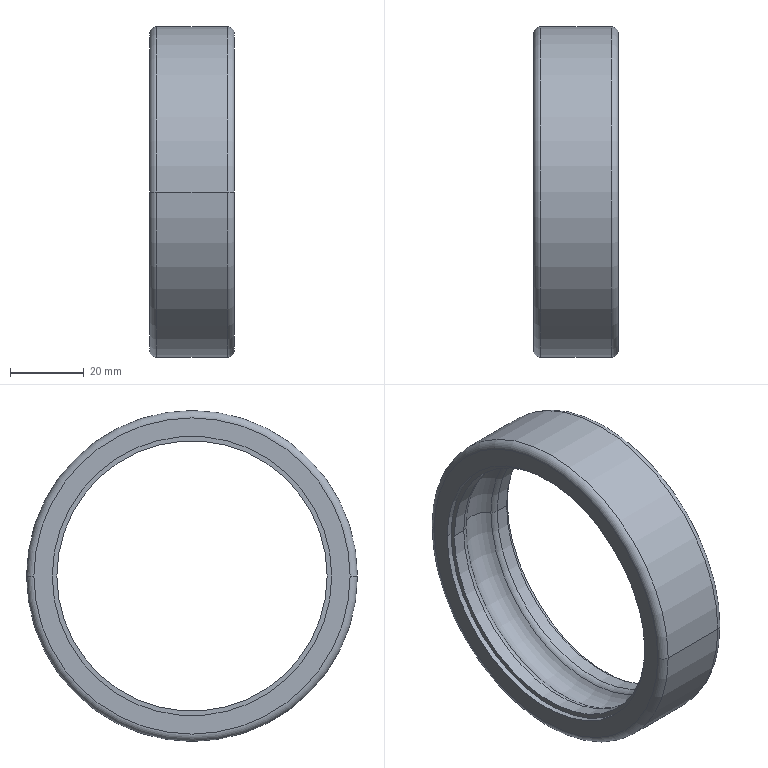Component | SolidWorks | 6308-OuterRing-1 | 1 solid | 24 faces | box 23.1 x 90 x 90 mm | volume 41581 mm3 | torus 10 | cylinder 10 | plane 4 | commonest cylinder face diameters 76 x4 73.5 x4 90 x2 | material AISI 304
build123d program:
from build123d import *

# Parameters (mm, degrees)
SKETCH1_R           = 45
SKETCH1_R_2         = 36.75
BOSS_EXTRUDE1_DEPTH = 11.55
FILLET1_R           = 2
SKETCH2_R           = 38
CUT_EXTRUDE1_DEPTH  = 1.5
SKETCH3_R           = 6
FILLET2_R           = 2


with BuildPart() as part:
    # Sketch1 → Boss-Extrude1 (new, symmetric)
    with BuildSketch(Plane.XY):
        Circle(SKETCH1_R)
        Circle(SKETCH1_R_2, mode=Mode.SUBTRACT)
    extrude(amount=BOSS_EXTRUDE1_DEPTH, both=True)

    # Fillet1
    fillet1_edges = [part.edges().sort_by_distance(p)[0] for p in [
        (-45, 0, -11.55),
        (-45, 0, 11.55),
    ]]
    fillet(fillet1_edges, radius=FILLET1_R)

    # Sketch2 → Cut-Extrude1 (cut)
    with BuildSketch(Plane.XY.offset(11.55)):
        Circle(SKETCH2_R)
    cut_extrude1 = extrude(amount=-CUT_EXTRUDE1_DEPTH, mode=Mode.SUBTRACT)

    # Mirror1: Cut-Extrude1 across plane
    add(cut_extrude1.mirror(Plane.XY), mode=Mode.SUBTRACT)

    # Sketch3 → Cut-Revolve1 (revolve, cut)
    with BuildSketch(Plane(origin=(0, 0, 0), x_dir=(0, 0, -1), z_dir=(1, 0, 0)), mode=Mode.PRIVATE) as cut_revolve1_sk:
        with Locations((0, 34)):
            Circle(SKETCH3_R)
    revolve(cut_revolve1_sk.sketch.rotate(Axis((0, 0, -32.915), (0, 0, 1)), 90), axis=Axis((0, 0, -32.915), (0, 0, 1)), mode=Mode.SUBTRACT)

    # Fillet2
    fillet2_edges = [part.edges().sort_by_distance(p)[0] for p in [
        (0, 36.75, 5.333),
        (0, -36.75, -5.333),
    ]]
    fillet(fillet2_edges, radius=FILLET2_R)


solid = part.part

# Placed as in the assembly
solid = solid.moved(Location((0, 136.117, 0), (0, 90, 0)))
STEP:
#1=COLOUR_RGB('',0.7922,0.8196,0.9333);
#2=FILL_AREA_STYLE_COLOUR('',#1);
#3=FILL_AREA_STYLE('',(#2));
#4=SURFACE_STYLE_FILL_AREA(#3);
#5=SURFACE_SIDE_STYLE('',(#4));
#6=SURFACE_STYLE_USAGE(.BOTH.,#5);
#7=PRESENTATION_STYLE_ASSIGNMENT((#6));
#8=CARTESIAN_POINT('',(0.1901,3.88,-0.));
#9=VERTEX_POINT('',#8);
#10=CARTESIAN_POINT('',(0.1901,6.838,-0.));
#11=VERTEX_POINT('',#10);
#12=CARTESIAN_POINT('',(0.1901,5.359,-0.));
#13=DIRECTION('',(1.,0.,0.));
#14=DIRECTION('',(-0.,1.,0.));
#15=AXIS2_PLACEMENT_3D('',#12,#13,#14);
#16=CIRCLE('',#15,1.479);
#17=EDGE_CURVE('',#9,#11,#16,.T.);
#18=ORIENTED_EDGE('',*,*,#17,.F.);
#19=CARTESIAN_POINT('',(0.2534,3.912,-0.));
#20=VERTEX_POINT('',#19);
#21=CARTESIAN_POINT('',(0.2534,3.833,-0.));
#22=DIRECTION('',(-0.,0.,-1.));
#23=DIRECTION('',(0.,1.,0.));
#24=AXIS2_PLACEMENT_3D('',#21,#22,#23);
#25=CIRCLE('',#24,0.07874);
#26=EDGE_CURVE('',#9,#20,#25,.T.);
#27=ORIENTED_EDGE('',*,*,#26,.T.);
#28=CARTESIAN_POINT('',(0.2534,6.806,-0.));
#29=VERTEX_POINT('',#28);
#30=CARTESIAN_POINT('',(0.2534,5.359,-0.));
#31=DIRECTION('',(-1.,-0.,-0.));
#32=DIRECTION('',(-0.,1.,0.));
#33=AXIS2_PLACEMENT_3D('',#30,#31,#32);
#34=CIRCLE('',#33,1.447);
#35=EDGE_CURVE('',#29,#20,#34,.T.);
#36=ORIENTED_EDGE('',*,*,#35,.F.);
#37=CARTESIAN_POINT('',(0.2534,6.885,-0.));
#38=DIRECTION('',(0.,-0.,1.));
#39=DIRECTION('',(0.,-1.,-0.));
#40=AXIS2_PLACEMENT_3D('',#37,#38,#39);
#41=CIRCLE('',#40,0.07874);
#42=EDGE_CURVE('',#11,#29,#41,.T.);
#43=ORIENTED_EDGE('',*,*,#42,.F.);
#44=EDGE_LOOP('',(#18,#27,#36,#43));
#45=FACE_OUTER_BOUND('',#44,.T.);
#46=CARTESIAN_POINT('',(0.2534,5.359,-0.));
#47=DIRECTION('',(-1.,-0.,-0.));
#48=DIRECTION('',(-0.,1.,0.));
#49=AXIS2_PLACEMENT_3D('',#46,#47,#48);
#50=TOROIDAL_SURFACE('',#49,1.526,0.07874);
#51=ADVANCED_FACE('',(#45),#50,.T.);
#52=CARTESIAN_POINT('',(-0.1901,6.838,-0.));
#53=VERTEX_POINT('',#52);
#54=CARTESIAN_POINT('',(-0.1901,3.88,-0.));
#55=VERTEX_POINT('',#54);
#56=CARTESIAN_POINT('',(-0.1901,5.359,-0.));
#57=DIRECTION('',(-1.,-0.,-0.));
#58=DIRECTION('',(0.,-1.,-0.));
#59=AXIS2_PLACEMENT_3D('',#56,#57,#58);
#60=CIRCLE('',#59,1.479);
#61=EDGE_CURVE('',#53,#55,#60,.T.);
#62=ORIENTED_EDGE('',*,*,#61,.F.);
#63=CARTESIAN_POINT('',(-0.2534,6.806,-0.));
#64=VERTEX_POINT('',#63);
#65=CARTESIAN_POINT('',(-0.2534,6.885,-0.));
#66=DIRECTION('',(0.,-0.,-1.));
#67=DIRECTION('',(0.,1.,-0.));
#68=AXIS2_PLACEMENT_3D('',#65,#66,#67);
#69=CIRCLE('',#68,0.07874);
#70=EDGE_CURVE('',#53,#64,#69,.T.);
#71=ORIENTED_EDGE('',*,*,#70,.T.);
#72=CARTESIAN_POINT('',(-0.2534,3.912,-0.));
#73=VERTEX_POINT('',#72);
#74=CARTESIAN_POINT('',(-0.2534,5.359,-0.));
#75=DIRECTION('',(1.,0.,0.));
#76=DIRECTION('',(0.,-1.,-0.));
#77=AXIS2_PLACEMENT_3D('',#74,#75,#76);
#78=CIRCLE('',#77,1.447);
#79=EDGE_CURVE('',#73,#64,#78,.T.);
#80=ORIENTED_EDGE('',*,*,#79,.F.);
#81=CARTESIAN_POINT('',(-0.2534,3.833,-0.));
#82=DIRECTION('',(0.,-0.,1.));
#83=DIRECTION('',(0.,-1.,-0.));
#84=AXIS2_PLACEMENT_3D('',#81,#82,#83);
#85=CIRCLE('',#84,0.07874);
#86=EDGE_CURVE('',#55,#73,#85,.T.);
#87=ORIENTED_EDGE('',*,*,#86,.F.);
#88=EDGE_LOOP('',(#62,#71,#80,#87));
#89=FACE_OUTER_BOUND('',#88,.T.);
#90=CARTESIAN_POINT('',(-0.2534,5.359,-0.));
#91=DIRECTION('',(1.,0.,0.));
#92=DIRECTION('',(0.,-1.,-0.));
#93=AXIS2_PLACEMENT_3D('',#90,#91,#92);
#94=TOROIDAL_SURFACE('',#93,1.526,0.07874);
#95=ADVANCED_FACE('',(#89),#94,.T.);
#96=CARTESIAN_POINT('',(0.1901,5.359,-0.));
#97=DIRECTION('',(1.,0.,0.));
#98=DIRECTION('',(-0.,1.,0.));
#99=AXIS2_PLACEMENT_3D('',#96,#97,#98);
#100=CIRCLE('',#99,1.479);
#101=EDGE_CURVE('',#11,#9,#100,.T.);
#102=ORIENTED_EDGE('',*,*,#101,.T.);
#103=CARTESIAN_POINT('',(-0.,4.02,-0.));
#104=DIRECTION('',(-0.,0.,-1.));
#105=DIRECTION('',(0.,1.,0.));
#106=AXIS2_PLACEMENT_3D('',#103,#104,#105);
#107=CIRCLE('',#106,0.2362);
#108=EDGE_CURVE('',#9,#55,#107,.T.);
#109=ORIENTED_EDGE('',*,*,#108,.T.);
#110=CARTESIAN_POINT('',(-0.1901,5.359,-0.));
#111=DIRECTION('',(-1.,-0.,-0.));
#112=DIRECTION('',(0.,-1.,-0.));
#113=AXIS2_PLACEMENT_3D('',#110,#111,#112);
#114=CIRCLE('',#113,1.479);
#115=EDGE_CURVE('',#55,#53,#114,.T.);
#116=ORIENTED_EDGE('',*,*,#115,.T.);
#117=CARTESIAN_POINT('',(-0.,6.698,-0.));
#118=DIRECTION('',(0.,-0.,1.));
#119=DIRECTION('',(0.,-1.,-0.));
#120=AXIS2_PLACEMENT_3D('',#117,#118,#119);
#121=CIRCLE('',#120,0.2362);
#122=EDGE_CURVE('',#11,#53,#121,.T.);
#123=ORIENTED_EDGE('',*,*,#122,.F.);
#124=EDGE_LOOP('',(#102,#109,#116,#123));
#125=FACE_OUTER_BOUND('',#124,.T.);
#126=CARTESIAN_POINT('',(-0.,5.359,-0.));
#127=DIRECTION('',(-1.,-0.,-0.));
#128=DIRECTION('',(-0.,1.,0.));
#129=AXIS2_PLACEMENT_3D('',#126,#127,#128);
#130=TOROIDAL_SURFACE('',#129,1.339,0.2362);
#131=ADVANCED_FACE('',(#125),#130,.F.);
#132=CARTESIAN_POINT('',(-0.3957,6.855,-0.));
#133=VERTEX_POINT('',#132);
#134=CARTESIAN_POINT('',(-0.3957,3.863,-0.));
#135=VERTEX_POINT('',#134);
#136=CARTESIAN_POINT('',(-0.3957,5.359,-0.));
#137=DIRECTION('',(1.,0.,0.));
#138=DIRECTION('',(0.,-1.,-0.));
#139=AXIS2_PLACEMENT_3D('',#136,#137,#138);
#140=CIRCLE('',#139,1.496);
#141=EDGE_CURVE('',#133,#135,#140,.T.);
#142=ORIENTED_EDGE('',*,*,#141,.T.);
#143=CARTESIAN_POINT('',(-0.4547,3.863,-0.));
#144=VERTEX_POINT('',#143);
#145=CARTESIAN_POINT('',(-0.3957,3.863,-0.));
#146=DIRECTION('',(-1.,-0.,-0.));
#147=VECTOR('',#146,39.37);
#148=LINE('',#145,#147);
#149=EDGE_CURVE('',#135,#144,#148,.T.);
#150=ORIENTED_EDGE('',*,*,#149,.T.);
#151=CARTESIAN_POINT('',(-0.4547,6.855,-0.));
#152=VERTEX_POINT('',#151);
#153=CARTESIAN_POINT('',(-0.4547,5.359,-0.));
#154=DIRECTION('',(1.,0.,0.));
#155=DIRECTION('',(0.,-1.,-0.));
#156=AXIS2_PLACEMENT_3D('',#153,#154,#155);
#157=CIRCLE('',#156,1.496);
#158=EDGE_CURVE('',#152,#144,#157,.T.);
#159=ORIENTED_EDGE('',*,*,#158,.F.);
#160=CARTESIAN_POINT('',(-0.3957,6.855,-0.));
#161=DIRECTION('',(-1.,-0.,-0.));
#162=VECTOR('',#161,39.37);
#163=LINE('',#160,#162);
#164=EDGE_CURVE('',#133,#152,#163,.T.);
#165=ORIENTED_EDGE('',*,*,#164,.F.);
#166=EDGE_LOOP('',(#142,#150,#159,#165));
#167=FACE_OUTER_BOUND('',#166,.T.);
#168=CARTESIAN_POINT('',(-0.3957,5.359,-0.));
#169=DIRECTION('',(-1.,-0.,-0.));
#170=DIRECTION('',(-0.,1.,0.));
#171=AXIS2_PLACEMENT_3D('',#168,#169,#170);
#172=CYLINDRICAL_SURFACE('',#171,1.496);
#173=ADVANCED_FACE('',(#167),#172,.F.);
#174=CARTESIAN_POINT('',(0.3957,6.855,-0.));
#175=VERTEX_POINT('',#174);
#176=CARTESIAN_POINT('',(0.3957,3.863,-0.));
#177=VERTEX_POINT('',#176);
#178=CARTESIAN_POINT('',(0.3957,5.359,-0.));
#179=DIRECTION('',(1.,0.,0.));
#180=DIRECTION('',(0.,-1.,-0.));
#181=AXIS2_PLACEMENT_3D('',#178,#179,#180);
#182=CIRCLE('',#181,1.496);
#183=EDGE_CURVE('',#175,#177,#182,.T.);
#184=ORIENTED_EDGE('',*,*,#183,.F.);
#185=CARTESIAN_POINT('',(0.4547,6.855,-0.));
#186=VERTEX_POINT('',#185);
#187=CARTESIAN_POINT('',(0.3957,6.855,-0.));
#188=DIRECTION('',(1.,0.,0.));
#189=VECTOR('',#188,39.37);
#190=LINE('',#187,#189);
#191=EDGE_CURVE('',#175,#186,#190,.T.);
#192=ORIENTED_EDGE('',*,*,#191,.T.);
#193=CARTESIAN_POINT('',(0.4547,3.863,-0.));
#194=VERTEX_POINT('',#193);
#195=CARTESIAN_POINT('',(0.4547,5.359,-0.));
#196=DIRECTION('',(1.,0.,0.));
#197=DIRECTION('',(0.,-1.,-0.));
#198=AXIS2_PLACEMENT_3D('',#195,#196,#197);
#199=CIRCLE('',#198,1.496);
#200=EDGE_CURVE('',#186,#194,#199,.T.);
#201=ORIENTED_EDGE('',*,*,#200,.T.);
#202=CARTESIAN_POINT('',(0.3957,3.863,-0.));
#203=DIRECTION('',(1.,0.,0.));
#204=VECTOR('',#203,39.37);
#205=LINE('',#202,#204);
#206=EDGE_CURVE('',#177,#194,#205,.T.);
#207=ORIENTED_EDGE('',*,*,#206,.F.);
#208=EDGE_LOOP('',(#184,#192,#201,#207));
#209=FACE_OUTER_BOUND('',#208,.T.);
#210=CARTESIAN_POINT('',(0.3957,5.359,-0.));
#211=DIRECTION('',(1.,0.,0.));
#212=DIRECTION('',(0.,-1.,-0.));
#213=AXIS2_PLACEMENT_3D('',#210,#211,#212);
#214=CYLINDRICAL_SURFACE('',#213,1.496);
#215=ADVANCED_FACE('',(#209),#214,.F.);
#216=CARTESIAN_POINT('',(0.376,7.131,-0.));
#217=VERTEX_POINT('',#216);
#218=CARTESIAN_POINT('',(0.376,3.587,-0.));
#219=VERTEX_POINT('',#218);
#220=CARTESIAN_POINT('',(0.376,5.359,-0.));
#221=DIRECTION('',(-1.,-0.,-0.));
#222=DIRECTION('',(0.,-1.,-0.));
#223=AXIS2_PLACEMENT_3D('',#220,#221,#222);
#224=CIRCLE('',#223,1.772);
#225=EDGE_CURVE('',#217,#219,#224,.T.);
#226=ORIENTED_EDGE('',*,*,#225,.F.);
#227=CARTESIAN_POINT('',(0.4547,7.052,-0.));
#228=VERTEX_POINT('',#227);
#229=CARTESIAN_POINT('',(0.376,7.052,-0.));
#230=DIRECTION('',(0.,-0.,-1.));
#231=DIRECTION('',(0.,1.,-0.));
#232=AXIS2_PLACEMENT_3D('',#229,#230,#231);
#233=CIRCLE('',#232,0.07874);
#234=EDGE_CURVE('',#217,#228,#233,.T.);
#235=ORIENTED_EDGE('',*,*,#234,.T.);
#236=CARTESIAN_POINT('',(0.4547,3.666,-0.));
#237=VERTEX_POINT('',#236);
#238=CARTESIAN_POINT('',(0.4547,5.359,-0.));
#239=DIRECTION('',(1.,0.,0.));
#240=DIRECTION('',(0.,-1.,-0.));
#241=AXIS2_PLACEMENT_3D('',#238,#239,#240);
#242=CIRCLE('',#241,1.693);
#243=EDGE_CURVE('',#237,#228,#242,.T.);
#244=ORIENTED_EDGE('',*,*,#243,.F.);
#245=CARTESIAN_POINT('',(0.376,3.666,-0.));
#246=DIRECTION('',(0.,-0.,1.));
#247=DIRECTION('',(0.,-1.,-0.));
#248=AXIS2_PLACEMENT_3D('',#245,#246,#247);
#249=CIRCLE('',#248,0.07874);
#250=EDGE_CURVE('',#219,#237,#249,.T.);
#251=ORIENTED_EDGE('',*,*,#250,.F.);
#252=EDGE_LOOP('',(#226,#235,#244,#251));
#253=FACE_OUTER_BOUND('',#252,.T.);
#254=CARTESIAN_POINT('',(0.376,5.359,-0.));
#255=DIRECTION('',(1.,0.,0.));
#256=DIRECTION('',(0.,-1.,-0.));
#257=AXIS2_PLACEMENT_3D('',#254,#255,#256);
#258=TOROIDAL_SURFACE('',#257,1.693,0.07874);
#259=ADVANCED_FACE('',(#253),#258,.T.);
#260=CARTESIAN_POINT('',(-0.4547,7.052,-0.));
#261=VERTEX_POINT('',#260);
#262=CARTESIAN_POINT('',(-0.4547,3.666,-0.));
#263=VERTEX_POINT('',#262);
#264=CARTESIAN_POINT('',(-0.4547,5.359,-0.));
#265=DIRECTION('',(-1.,-0.,-0.));
#266=DIRECTION('',(0.,-1.,-0.));
#267=AXIS2_PLACEMENT_3D('',#264,#265,#266);
#268=CIRCLE('',#267,1.693);
#269=EDGE_CURVE('',#261,#263,#268,.T.);
#270=ORIENTED_EDGE('',*,*,#269,.F.);
#271=CARTESIAN_POINT('',(-0.376,7.131,-0.));
#272=VERTEX_POINT('',#271);
#273=CARTESIAN_POINT('',(-0.376,7.052,-0.));
#274=DIRECTION('',(0.,-0.,-1.));
#275=DIRECTION('',(0.,1.,-0.));
#276=AXIS2_PLACEMENT_3D('',#273,#274,#275);
#277=CIRCLE('',#276,0.07874);
#278=EDGE_CURVE('',#261,#272,#277,.T.);
#279=ORIENTED_EDGE('',*,*,#278,.T.);
#280=CARTESIAN_POINT('',(-0.376,3.587,-0.));
#281=VERTEX_POINT('',#280);
#282=CARTESIAN_POINT('',(-0.376,5.359,-0.));
#283=DIRECTION('',(1.,0.,0.));
#284=DIRECTION('',(0.,-1.,-0.));
#285=AXIS2_PLACEMENT_3D('',#282,#283,#284);
#286=CIRCLE('',#285,1.772);
#287=EDGE_CURVE('',#281,#272,#286,.T.);
#288=ORIENTED_EDGE('',*,*,#287,.F.);
#289=CARTESIAN_POINT('',(-0.376,3.666,-0.));
#290=DIRECTION('',(0.,-0.,1.));
#291=DIRECTION('',(0.,-1.,-0.));
#292=AXIS2_PLACEMENT_3D('',#289,#290,#291);
#293=CIRCLE('',#292,0.07874);
#294=EDGE_CURVE('',#263,#281,#293,.T.);
#295=ORIENTED_EDGE('',*,*,#294,.F.);
#296=EDGE_LOOP('',(#270,#279,#288,#295));
#297=FACE_OUTER_BOUND('',#296,.T.);
#298=CARTESIAN_POINT('',(-0.376,5.359,-0.));
#299=DIRECTION('',(1.,0.,0.));
#300=DIRECTION('',(0.,-1.,-0.));
#301=AXIS2_PLACEMENT_3D('',#298,#299,#300);
#302=TOROIDAL_SURFACE('',#301,1.693,0.07874);
#303=ADVANCED_FACE('',(#297),#302,.T.);
#304=ORIENTED_EDGE('',*,*,#225,.T.);
#305=CARTESIAN_POINT('',(0.4547,3.587,-0.));
#306=DIRECTION('',(-1.,-0.,-0.));
#307=VECTOR('',#306,39.37);
#308=LINE('',#305,#307);
#309=EDGE_CURVE('',#219,#281,#308,.T.);
#310=ORIENTED_EDGE('',*,*,#309,.T.);
#311=ORIENTED_EDGE('',*,*,#287,.T.);
#312=CARTESIAN_POINT('',(0.4547,7.131,-0.));
#313=DIRECTION('',(-1.,-0.,-0.));
#314=VECTOR('',#313,39.37);
#315=LINE('',#312,#314);
#316=EDGE_CURVE('',#217,#272,#315,.T.);
#317=ORIENTED_EDGE('',*,*,#316,.F.);
#318=EDGE_LOOP('',(#304,#310,#311,#317));
#319=FACE_OUTER_BOUND('',#318,.T.);
#320=CARTESIAN_POINT('',(0.4547,5.359,-0.));
#321=DIRECTION('',(-1.,-0.,-0.));
#322=DIRECTION('',(-0.,1.,0.));
#323=AXIS2_PLACEMENT_3D('',#320,#321,#322);
#324=CYLINDRICAL_SURFACE('',#323,1.772);
#325=ADVANCED_FACE('',(#319),#324,.T.);
#326=CARTESIAN_POINT('',(0.3957,6.806,-0.));
#327=VERTEX_POINT('',#326);
#328=CARTESIAN_POINT('',(0.3957,3.912,-0.));
#329=VERTEX_POINT('',#328);
#330=CARTESIAN_POINT('',(0.3957,5.359,-0.));
#331=DIRECTION('',(1.,0.,0.));
#332=DIRECTION('',(0.,-1.,-0.));
#333=AXIS2_PLACEMENT_3D('',#330,#331,#332);
#334=CIRCLE('',#333,1.447);
#335=EDGE_CURVE('',#327,#329,#334,.T.);
#336=ORIENTED_EDGE('',*,*,#335,.T.);
#337=CARTESIAN_POINT('',(0.4547,3.912,-0.));
#338=DIRECTION('',(-1.,-0.,-0.));
#339=VECTOR('',#338,39.37);
#340=LINE('',#337,#339);
#341=EDGE_CURVE('',#329,#20,#340,.T.);
#342=ORIENTED_EDGE('',*,*,#341,.T.);
#343=CARTESIAN_POINT('',(0.2534,5.359,-0.));
#344=DIRECTION('',(-1.,-0.,-0.));
#345=DIRECTION('',(-0.,1.,0.));
#346=AXIS2_PLACEMENT_3D('',#343,#344,#345);
#347=CIRCLE('',#346,1.447);
#348=EDGE_CURVE('',#20,#29,#347,.T.);
#349=ORIENTED_EDGE('',*,*,#348,.T.);
#350=CARTESIAN_POINT('',(0.4547,6.806,-0.));
#351=DIRECTION('',(-1.,-0.,-0.));
#352=VECTOR('',#351,39.37);
#353=LINE('',#350,#352);
#354=EDGE_CURVE('',#327,#29,#353,.T.);
#355=ORIENTED_EDGE('',*,*,#354,.F.);
#356=EDGE_LOOP('',(#336,#342,#349,#355));
#357=FACE_OUTER_BOUND('',#356,.T.);
#358=CARTESIAN_POINT('',(0.4547,5.359,-0.));
#359=DIRECTION('',(-1.,-0.,-0.));
#360=DIRECTION('',(-0.,1.,0.));
#361=AXIS2_PLACEMENT_3D('',#358,#359,#360);
#362=CYLINDRICAL_SURFACE('',#361,1.447);
#363=ADVANCED_FACE('',(#357),#362,.F.);
#364=CARTESIAN_POINT('',(-0.2534,5.359,-0.));
#365=DIRECTION('',(1.,0.,0.));
#366=DIRECTION('',(0.,-1.,-0.));
#367=AXIS2_PLACEMENT_3D('',#364,#365,#366);
#368=CIRCLE('',#367,1.447);
#369=EDGE_CURVE('',#64,#73,#368,.T.);
#370=ORIENTED_EDGE('',*,*,#369,.T.);
#371=CARTESIAN_POINT('',(-0.3957,3.912,-0.));
#372=VERTEX_POINT('',#371);
#373=CARTESIAN_POINT('',(0.4547,3.912,-0.));
#374=DIRECTION('',(-1.,-0.,-0.));
#375=VECTOR('',#374,39.37);
#376=LINE('',#373,#375);
#377=EDGE_CURVE('',#73,#372,#376,.T.);
#378=ORIENTED_EDGE('',*,*,#377,.T.);
#379=CARTESIAN_POINT('',(-0.3957,6.806,-0.));
#380=VERTEX_POINT('',#379);
#381=CARTESIAN_POINT('',(-0.3957,5.359,-0.));
#382=DIRECTION('',(-1.,-0.,-0.));
#383=DIRECTION('',(-0.,1.,0.));
#384=AXIS2_PLACEMENT_3D('',#381,#382,#383);
#385=CIRCLE('',#384,1.447);
#386=EDGE_CURVE('',#372,#380,#385,.T.);
#387=ORIENTED_EDGE('',*,*,#386,.T.);
#388=CARTESIAN_POINT('',(0.4547,6.806,-0.));
#389=DIRECTION('',(-1.,-0.,-0.));
#390=VECTOR('',#389,39.37);
#391=LINE('',#388,#390);
#392=EDGE_CURVE('',#64,#380,#391,.T.);
#393=ORIENTED_EDGE('',*,*,#392,.F.);
#394=EDGE_LOOP('',(#370,#378,#387,#393));
#395=FACE_OUTER_BOUND('',#394,.T.);
#396=CARTESIAN_POINT('',(0.4547,5.359,-0.));
#397=DIRECTION('',(-1.,-0.,-0.));
#398=DIRECTION('',(-0.,1.,0.));
#399=AXIS2_PLACEMENT_3D('',#396,#397,#398);
#400=CYLINDRICAL_SURFACE('',#399,1.447);
#401=ADVANCED_FACE('',(#395),#400,.F.);
#402=ORIENTED_EDGE('',*,*,#377,.F.);
#403=ORIENTED_EDGE('',*,*,#79,.T.);
#404=ORIENTED_EDGE('',*,*,#392,.T.);
#405=CARTESIAN_POINT('',(-0.3957,5.359,-0.));
#406=DIRECTION('',(-1.,-0.,-0.));
#407=DIRECTION('',(-0.,1.,0.));
#408=AXIS2_PLACEMENT_3D('',#405,#406,#407);
#409=CIRCLE('',#408,1.447);
#410=EDGE_CURVE('',#380,#372,#409,.T.);
#411=ORIENTED_EDGE('',*,*,#410,.T.);
#412=EDGE_LOOP('',(#402,#403,#404,#411));
#413=FACE_OUTER_BOUND('',#412,.T.);
#414=CARTESIAN_POINT('',(0.4547,5.359,-0.));
#415=DIRECTION('',(-1.,-0.,-0.));
#416=DIRECTION('',(-0.,1.,0.));
#417=AXIS2_PLACEMENT_3D('',#414,#415,#416);
#418=CYLINDRICAL_SURFACE('',#417,1.447);
#419=ADVANCED_FACE('',(#413),#418,.F.);
#420=ORIENTED_EDGE('',*,*,#341,.F.);
#421=CARTESIAN_POINT('',(0.3957,5.359,-0.));
#422=DIRECTION('',(1.,0.,0.));
#423=DIRECTION('',(0.,-1.,-0.));
#424=AXIS2_PLACEMENT_3D('',#421,#422,#423);
#425=CIRCLE('',#424,1.447);
#426=EDGE_CURVE('',#329,#327,#425,.T.);
#427=ORIENTED_EDGE('',*,*,#426,.T.);
#428=ORIENTED_EDGE('',*,*,#354,.T.);
#429=ORIENTED_EDGE('',*,*,#35,.T.);
#430=EDGE_LOOP('',(#420,#427,#428,#429));
#431=FACE_OUTER_BOUND('',#430,.T.);
#432=CARTESIAN_POINT('',(0.4547,5.359,-0.));
#433=DIRECTION('',(-1.,-0.,-0.));
#434=DIRECTION('',(-0.,1.,0.));
#435=AXIS2_PLACEMENT_3D('',#432,#433,#434);
#436=CYLINDRICAL_SURFACE('',#435,1.447);
#437=ADVANCED_FACE('',(#431),#436,.F.);
#438=CARTESIAN_POINT('',(0.4547,5.359,-0.));
#439=DIRECTION('',(1.,0.,0.));
#440=DIRECTION('',(0.,-1.,-0.));
#441=AXIS2_PLACEMENT_3D('',#438,#439,#440);
#442=CIRCLE('',#441,1.496);
#443=EDGE_CURVE('',#194,#186,#442,.T.);
#444=ORIENTED_EDGE('',*,*,#443,.F.);
#445=ORIENTED_EDGE('',*,*,#200,.F.);
#446=EDGE_LOOP('',(#444,#445));
#447=FACE_BOUND('',#446,.T.);
#448=ORIENTED_EDGE('',*,*,#243,.T.);
#449=CARTESIAN_POINT('',(0.4547,5.359,-0.));
#450=DIRECTION('',(1.,0.,0.));
#451=DIRECTION('',(0.,-1.,-0.));
#452=AXIS2_PLACEMENT_3D('',#449,#450,#451);
#453=CIRCLE('',#452,1.693);
#454=EDGE_CURVE('',#228,#237,#453,.T.);
#455=ORIENTED_EDGE('',*,*,#454,.T.);
#456=EDGE_LOOP('',(#448,#455));
#457=FACE_OUTER_BOUND('',#456,.T.);
#458=CARTESIAN_POINT('',(0.4547,5.359,-0.));
#459=DIRECTION('',(1.,0.,0.));
#460=DIRECTION('',(0.,-1.,-0.));
#461=AXIS2_PLACEMENT_3D('',#458,#459,#460);
#462=PLANE('',#461);
#463=ADVANCED_FACE('',(#447,#457),#462,.T.);
#464=ORIENTED_EDGE('',*,*,#158,.T.);
#465=CARTESIAN_POINT('',(-0.4547,5.359,-0.));
#466=DIRECTION('',(1.,0.,0.));
#467=DIRECTION('',(0.,-1.,-0.));
#468=AXIS2_PLACEMENT_3D('',#465,#466,#467);
#469=CIRCLE('',#468,1.496);
#470=EDGE_CURVE('',#144,#152,#469,.T.);
#471=ORIENTED_EDGE('',*,*,#470,.T.);
#472=EDGE_LOOP('',(#464,#471));
#473=FACE_BOUND('',#472,.T.);
#474=CARTESIAN_POINT('',(-0.4547,5.359,-0.));
#475=DIRECTION('',(-1.,-0.,-0.));
#476=DIRECTION('',(0.,-1.,-0.));
#477=AXIS2_PLACEMENT_3D('',#474,#475,#476);
#478=CIRCLE('',#477,1.693);
#479=EDGE_CURVE('',#263,#261,#478,.T.);
#480=ORIENTED_EDGE('',*,*,#479,.T.);
#481=ORIENTED_EDGE('',*,*,#269,.T.);
#482=EDGE_LOOP('',(#480,#481));
#483=FACE_OUTER_BOUND('',#482,.T.);
#484=CARTESIAN_POINT('',(-0.4547,5.359,-0.));
#485=DIRECTION('',(1.,0.,0.));
#486=DIRECTION('',(0.,-1.,-0.));
#487=AXIS2_PLACEMENT_3D('',#484,#485,#486);
#488=PLANE('',#487);
#489=ADVANCED_FACE('',(#473,#483),#488,.F.);
#490=ORIENTED_EDGE('',*,*,#309,.F.);
#491=CARTESIAN_POINT('',(0.376,5.359,-0.));
#492=DIRECTION('',(-1.,-0.,-0.));
#493=DIRECTION('',(0.,-1.,-0.));
#494=AXIS2_PLACEMENT_3D('',#491,#492,#493);
#495=CIRCLE('',#494,1.772);
#496=EDGE_CURVE('',#219,#217,#495,.T.);
#497=ORIENTED_EDGE('',*,*,#496,.T.);
#498=ORIENTED_EDGE('',*,*,#316,.T.);
#499=CARTESIAN_POINT('',(-0.376,5.359,-0.));
#500=DIRECTION('',(1.,0.,0.));
#501=DIRECTION('',(0.,-1.,-0.));
#502=AXIS2_PLACEMENT_3D('',#499,#500,#501);
#503=CIRCLE('',#502,1.772);
#504=EDGE_CURVE('',#272,#281,#503,.T.);
#505=ORIENTED_EDGE('',*,*,#504,.T.);
#506=EDGE_LOOP('',(#490,#497,#498,#505));
#507=FACE_OUTER_BOUND('',#506,.T.);
#508=CARTESIAN_POINT('',(0.4547,5.359,-0.));
#509=DIRECTION('',(-1.,-0.,-0.));
#510=DIRECTION('',(-0.,1.,0.));
#511=AXIS2_PLACEMENT_3D('',#508,#509,#510);
#512=CYLINDRICAL_SURFACE('',#511,1.772);
#513=ADVANCED_FACE('',(#507),#512,.T.);
#514=ORIENTED_EDGE('',*,*,#278,.F.);
#515=ORIENTED_EDGE('',*,*,#479,.F.);
#516=ORIENTED_EDGE('',*,*,#294,.T.);
#517=ORIENTED_EDGE('',*,*,#504,.F.);
#518=EDGE_LOOP('',(#514,#515,#516,#517));
#519=FACE_OUTER_BOUND('',#518,.T.);
#520=CARTESIAN_POINT('',(-0.376,5.359,-0.));
#521=DIRECTION('',(1.,0.,0.));
#522=DIRECTION('',(0.,-1.,-0.));
#523=AXIS2_PLACEMENT_3D('',#520,#521,#522);
#524=TOROIDAL_SURFACE('',#523,1.693,0.07874);
#525=ADVANCED_FACE('',(#519),#524,.T.);
#526=ORIENTED_EDGE('',*,*,#234,.F.);
#527=ORIENTED_EDGE('',*,*,#496,.F.);
#528=ORIENTED_EDGE('',*,*,#250,.T.);
#529=ORIENTED_EDGE('',*,*,#454,.F.);
#530=EDGE_LOOP('',(#526,#527,#528,#529));
#531=FACE_OUTER_BOUND('',#530,.T.);
#532=CARTESIAN_POINT('',(0.376,5.359,-0.));
#533=DIRECTION('',(1.,0.,0.));
#534=DIRECTION('',(0.,-1.,-0.));
#535=AXIS2_PLACEMENT_3D('',#532,#533,#534);
#536=TOROIDAL_SURFACE('',#535,1.693,0.07874);
#537=ADVANCED_FACE('',(#531),#536,.T.);
#538=ORIENTED_EDGE('',*,*,#191,.F.);
#539=CARTESIAN_POINT('',(0.3957,5.359,-0.));
#540=DIRECTION('',(1.,0.,0.));
#541=DIRECTION('',(0.,-1.,-0.));
#542=AXIS2_PLACEMENT_3D('',#539,#540,#541);
#543=CIRCLE('',#542,1.496);
#544=EDGE_CURVE('',#177,#175,#543,.T.);
#545=ORIENTED_EDGE('',*,*,#544,.F.);
#546=ORIENTED_EDGE('',*,*,#206,.T.);
#547=ORIENTED_EDGE('',*,*,#443,.T.);
#548=EDGE_LOOP('',(#538,#545,#546,#547));
#549=FACE_OUTER_BOUND('',#548,.T.);
#550=CARTESIAN_POINT('',(0.3957,5.359,-0.));
#551=DIRECTION('',(1.,0.,0.));
#552=DIRECTION('',(0.,-1.,-0.));
#553=AXIS2_PLACEMENT_3D('',#550,#551,#552);
#554=CYLINDRICAL_SURFACE('',#553,1.496);
#555=ADVANCED_FACE('',(#549),#554,.F.);
#556=ORIENTED_EDGE('',*,*,#335,.F.);
#557=ORIENTED_EDGE('',*,*,#426,.F.);
#558=EDGE_LOOP('',(#556,#557));
#559=FACE_BOUND('',#558,.T.);
#560=ORIENTED_EDGE('',*,*,#544,.T.);
#561=ORIENTED_EDGE('',*,*,#183,.T.);
#562=EDGE_LOOP('',(#560,#561));
#563=FACE_OUTER_BOUND('',#562,.T.);
#564=CARTESIAN_POINT('',(0.3957,5.359,-0.));
#565=DIRECTION('',(1.,0.,0.));
#566=DIRECTION('',(0.,-1.,-0.));
#567=AXIS2_PLACEMENT_3D('',#564,#565,#566);
#568=PLANE('',#567);
#569=ADVANCED_FACE('',(#559,#563),#568,.T.);
#570=ORIENTED_EDGE('',*,*,#149,.F.);
#571=CARTESIAN_POINT('',(-0.3957,5.359,-0.));
#572=DIRECTION('',(1.,0.,0.));
#573=DIRECTION('',(0.,-1.,-0.));
#574=AXIS2_PLACEMENT_3D('',#571,#572,#573);
#575=CIRCLE('',#574,1.496);
#576=EDGE_CURVE('',#135,#133,#575,.T.);
#577=ORIENTED_EDGE('',*,*,#576,.T.);
#578=ORIENTED_EDGE('',*,*,#164,.T.);
#579=ORIENTED_EDGE('',*,*,#470,.F.);
#580=EDGE_LOOP('',(#570,#577,#578,#579));
#581=FACE_OUTER_BOUND('',#580,.T.);
#582=CARTESIAN_POINT('',(-0.3957,5.359,-0.));
#583=DIRECTION('',(-1.,-0.,-0.));
#584=DIRECTION('',(-0.,1.,0.));
#585=AXIS2_PLACEMENT_3D('',#582,#583,#584);
#586=CYLINDRICAL_SURFACE('',#585,1.496);
#587=ADVANCED_FACE('',(#581),#586,.F.);
#588=ORIENTED_EDGE('',*,*,#410,.F.);
#589=ORIENTED_EDGE('',*,*,#386,.F.);
#590=EDGE_LOOP('',(#588,#589));
#591=FACE_BOUND('',#590,.T.);
#592=ORIENTED_EDGE('',*,*,#141,.F.);
#593=ORIENTED_EDGE('',*,*,#576,.F.);
#594=EDGE_LOOP('',(#592,#593));
#595=FACE_OUTER_BOUND('',#594,.T.);
#596=CARTESIAN_POINT('',(-0.3957,5.359,-0.));
#597=DIRECTION('',(-1.,-0.,-0.));
#598=DIRECTION('',(0.,-1.,-0.));
#599=AXIS2_PLACEMENT_3D('',#596,#597,#598);
#600=PLANE('',#599);
#601=ADVANCED_FACE('',(#591,#595),#600,.T.);
#602=ORIENTED_EDGE('',*,*,#108,.F.);
#603=ORIENTED_EDGE('',*,*,#17,.T.);
#604=ORIENTED_EDGE('',*,*,#122,.T.);
#605=ORIENTED_EDGE('',*,*,#61,.T.);
#606=EDGE_LOOP('',(#602,#603,#604,#605));
#607=FACE_OUTER_BOUND('',#606,.T.);
#608=CARTESIAN_POINT('',(-0.,5.359,-0.));
#609=DIRECTION('',(-1.,-0.,-0.));
#610=DIRECTION('',(-0.,1.,0.));
#611=AXIS2_PLACEMENT_3D('',#608,#609,#610);
#612=TOROIDAL_SURFACE('',#611,1.339,0.2362);
#613=ADVANCED_FACE('',(#607),#612,.F.);
#614=ORIENTED_EDGE('',*,*,#70,.F.);
#615=ORIENTED_EDGE('',*,*,#115,.F.);
#616=ORIENTED_EDGE('',*,*,#86,.T.);
#617=ORIENTED_EDGE('',*,*,#369,.F.);
#618=EDGE_LOOP('',(#614,#615,#616,#617));
#619=FACE_OUTER_BOUND('',#618,.T.);
#620=CARTESIAN_POINT('',(-0.2534,5.359,-0.));
#621=DIRECTION('',(1.,0.,0.));
#622=DIRECTION('',(0.,-1.,-0.));
#623=AXIS2_PLACEMENT_3D('',#620,#621,#622);
#624=TOROIDAL_SURFACE('',#623,1.526,0.07874);
#625=ADVANCED_FACE('',(#619),#624,.T.);
#626=ORIENTED_EDGE('',*,*,#26,.F.);
#627=ORIENTED_EDGE('',*,*,#101,.F.);
#628=ORIENTED_EDGE('',*,*,#42,.T.);
#629=ORIENTED_EDGE('',*,*,#348,.F.);
#630=EDGE_LOOP('',(#626,#627,#628,#629));
#631=FACE_OUTER_BOUND('',#630,.T.);
#632=CARTESIAN_POINT('',(0.2534,5.359,-0.));
#633=DIRECTION('',(-1.,-0.,-0.));
#634=DIRECTION('',(-0.,1.,0.));
#635=AXIS2_PLACEMENT_3D('',#632,#633,#634);
#636=TOROIDAL_SURFACE('',#635,1.526,0.07874);
#637=ADVANCED_FACE('',(#631),#636,.T.);
#638=CLOSED_SHELL('',(#51,#95,#131,#173,#215,#259,#303,#325,#363,#401,#419,#437,#463,#489,#513,#525,#537,#555,#569,#587,#601,#613,#625,#637));
#639=MANIFOLD_SOLID_BREP('',#638);
#640=STYLED_ITEM('',(#7),#639);
#641=(LENGTH_UNIT()NAMED_UNIT(*)SI_UNIT($,.METRE.));
#642=LENGTH_MEASURE_WITH_UNIT(LENGTH_MEASURE(0.0254),#641);
#643=DIMENSIONAL_EXPONENTS(1.,0.,0.,0.,0.,0.,0.);
#644=(CONVERSION_BASED_UNIT('',#642)LENGTH_UNIT()NAMED_UNIT(#643));
#645=UNCERTAINTY_MEASURE_WITH_UNIT(LENGTH_MEASURE(0.00001),#644,'','');
#646=(NAMED_UNIT(*)PLANE_ANGLE_UNIT()SI_UNIT($,.RADIAN.));
#647=(NAMED_UNIT(*)SI_UNIT($,.STERADIAN.)SOLID_ANGLE_UNIT());
#648=(GEOMETRIC_REPRESENTATION_CONTEXT(3)GLOBAL_UNCERTAINTY_ASSIGNED_CONTEXT((#645))GLOBAL_UNIT_ASSIGNED_CONTEXT((#644,#646,#647))REPRESENTATION_CONTEXT('',''));
#649=MECHANICAL_DESIGN_GEOMETRIC_PRESENTATION_REPRESENTATION('',(#640),#648);
#650=CARTESIAN_POINT('',(0.,0.,0.));
#651=DIRECTION('',(0.,0.,1.));
#652=DIRECTION('',(1.,0.,0.));
#653=AXIS2_PLACEMENT_3D('',#650,#651,#652);
#654=(LENGTH_UNIT()NAMED_UNIT(*)SI_UNIT($,.METRE.));
#655=LENGTH_MEASURE_WITH_UNIT(LENGTH_MEASURE(0.0254),#654);
#656=DIMENSIONAL_EXPONENTS(1.,0.,0.,0.,0.,0.,0.);
#657=(CONVERSION_BASED_UNIT('',#655)LENGTH_UNIT()NAMED_UNIT(#656));
#658=UNCERTAINTY_MEASURE_WITH_UNIT(LENGTH_MEASURE(0.00001),#657,'','');
#659=(NAMED_UNIT(*)PLANE_ANGLE_UNIT()SI_UNIT($,.RADIAN.));
#660=(NAMED_UNIT(*)SI_UNIT($,.STERADIAN.)SOLID_ANGLE_UNIT());
#661=(GEOMETRIC_REPRESENTATION_CONTEXT(3)GLOBAL_UNCERTAINTY_ASSIGNED_CONTEXT((#658))GLOBAL_UNIT_ASSIGNED_CONTEXT((#657,#659,#660))REPRESENTATION_CONTEXT('',''));
#662=ADVANCED_BREP_SHAPE_REPRESENTATION('',(#639,#653),#661);
#663=PRESENTATION_LAYER_ASSIGNMENT('','',(#640));